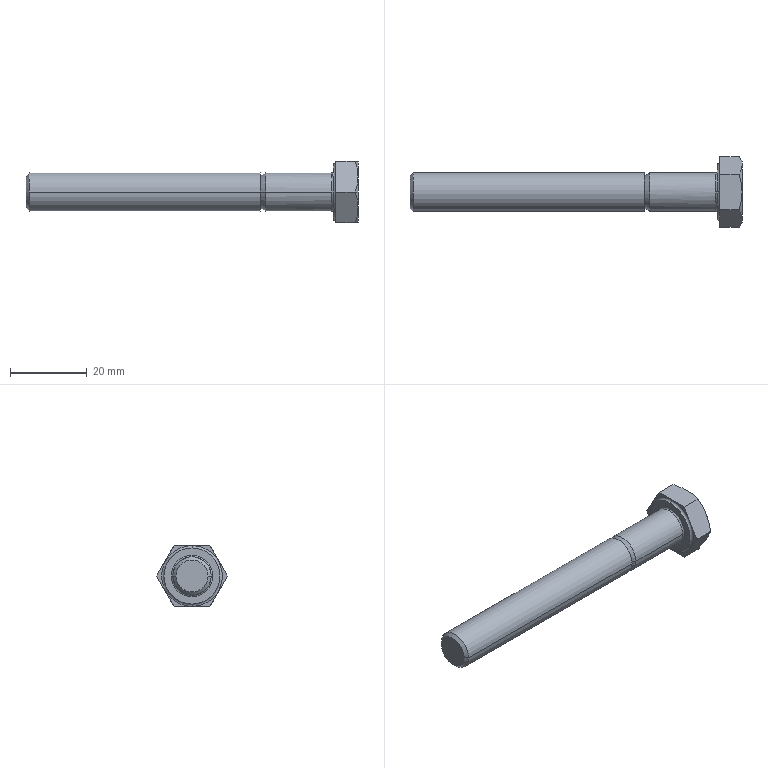Component | NX | M10X80 | 1 solid | 31 faces | volume 7643 mm3 | cone 12 | plane 11 | cylinder 4 | torus 4 | commonest cylinder face diameters 10 x4